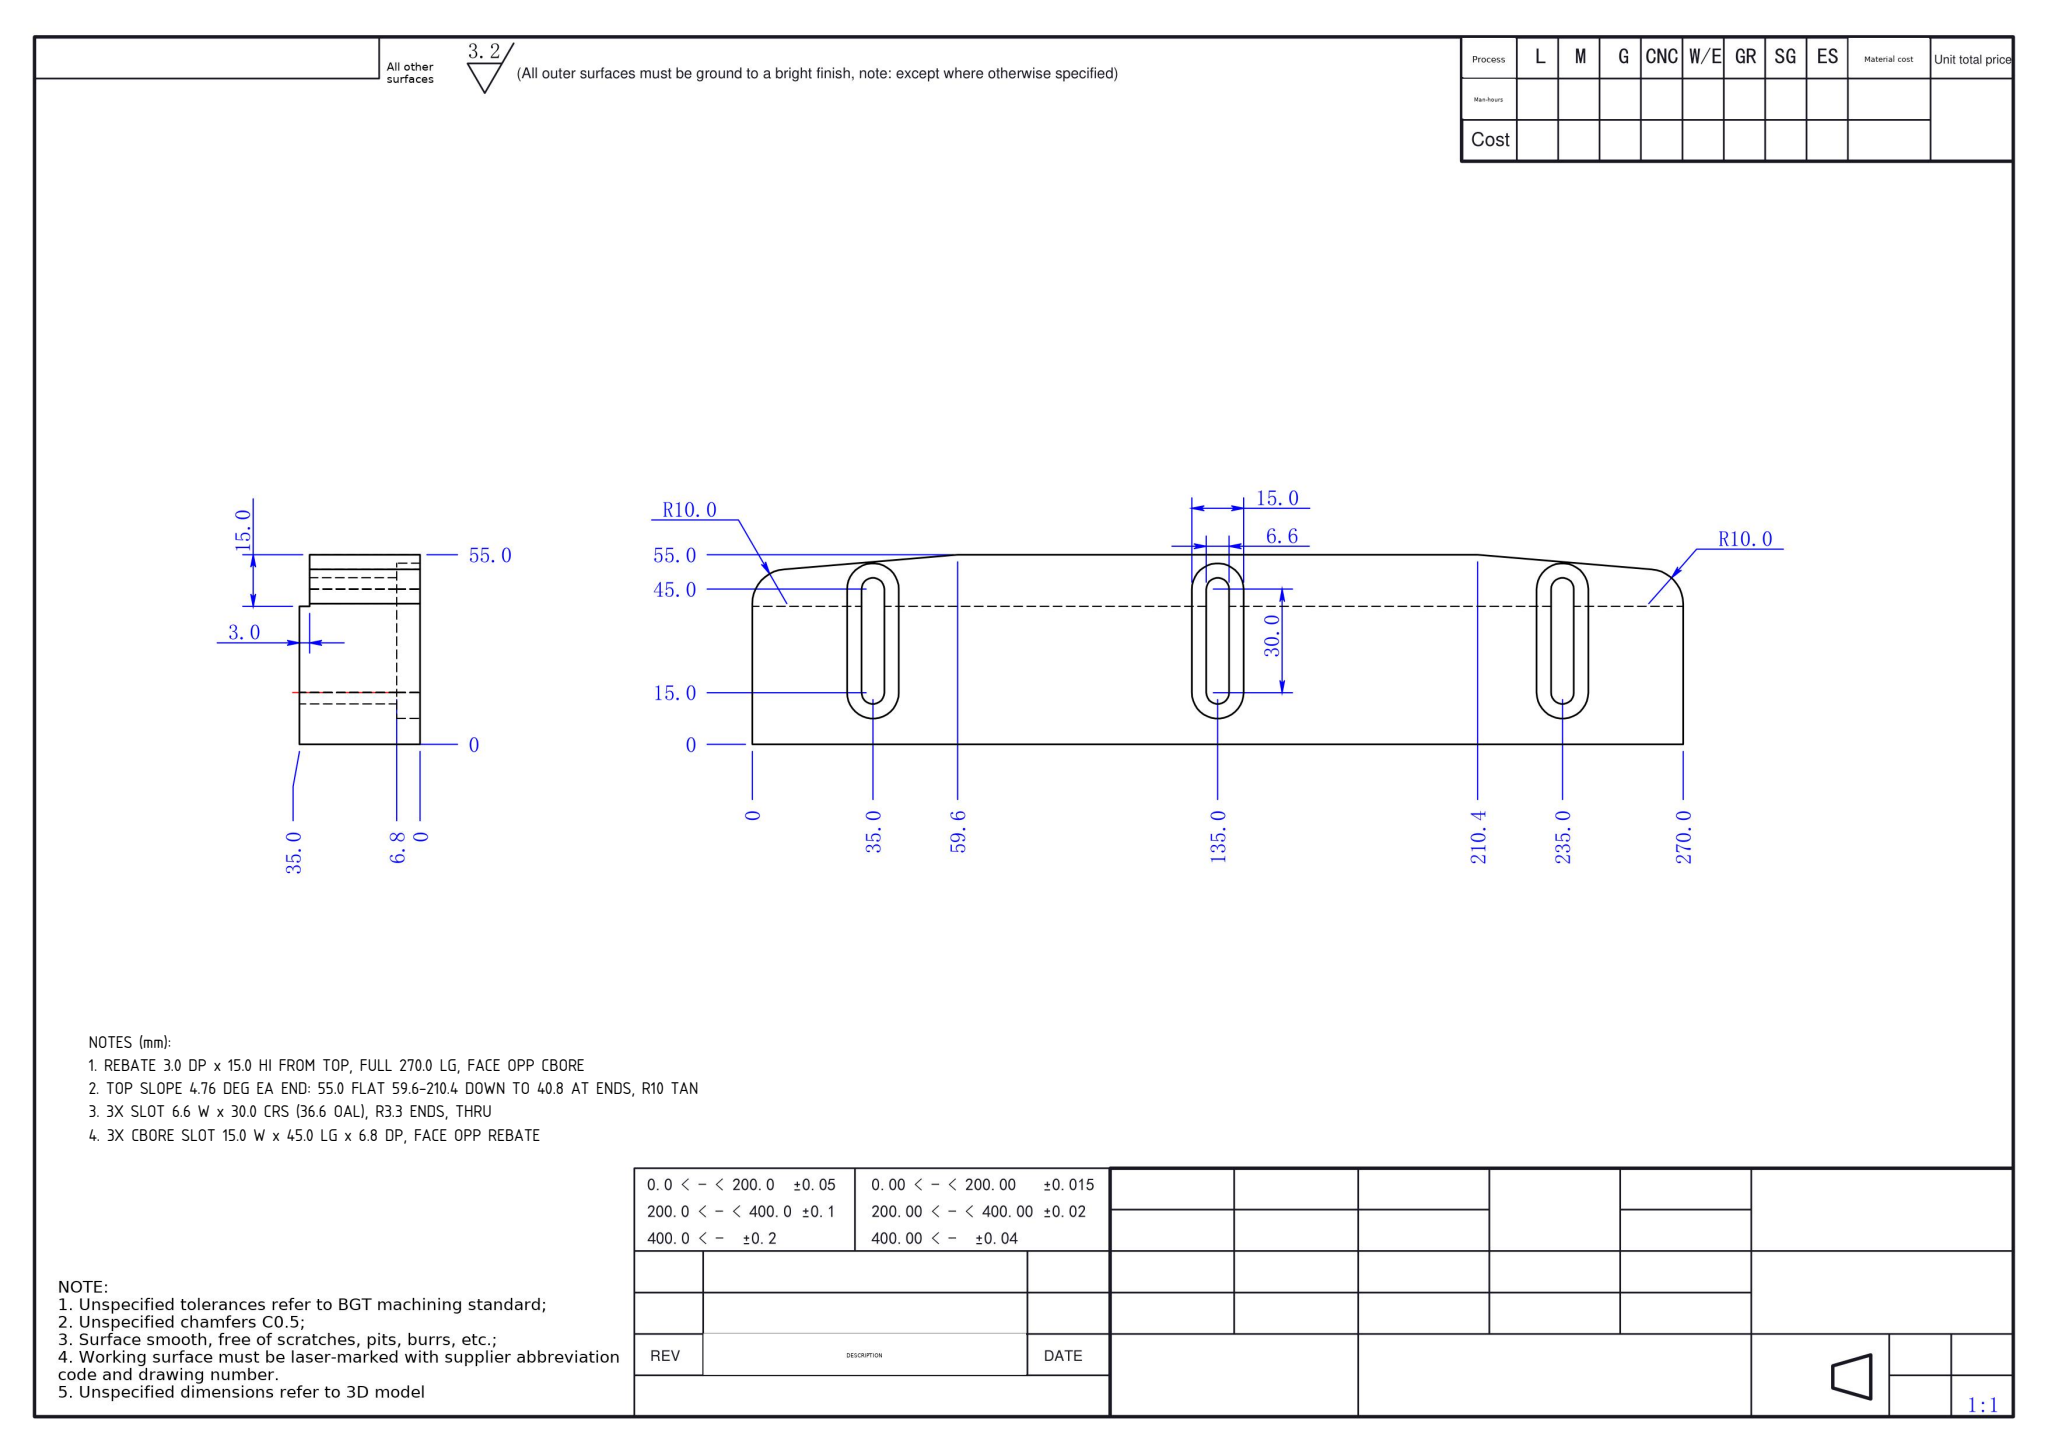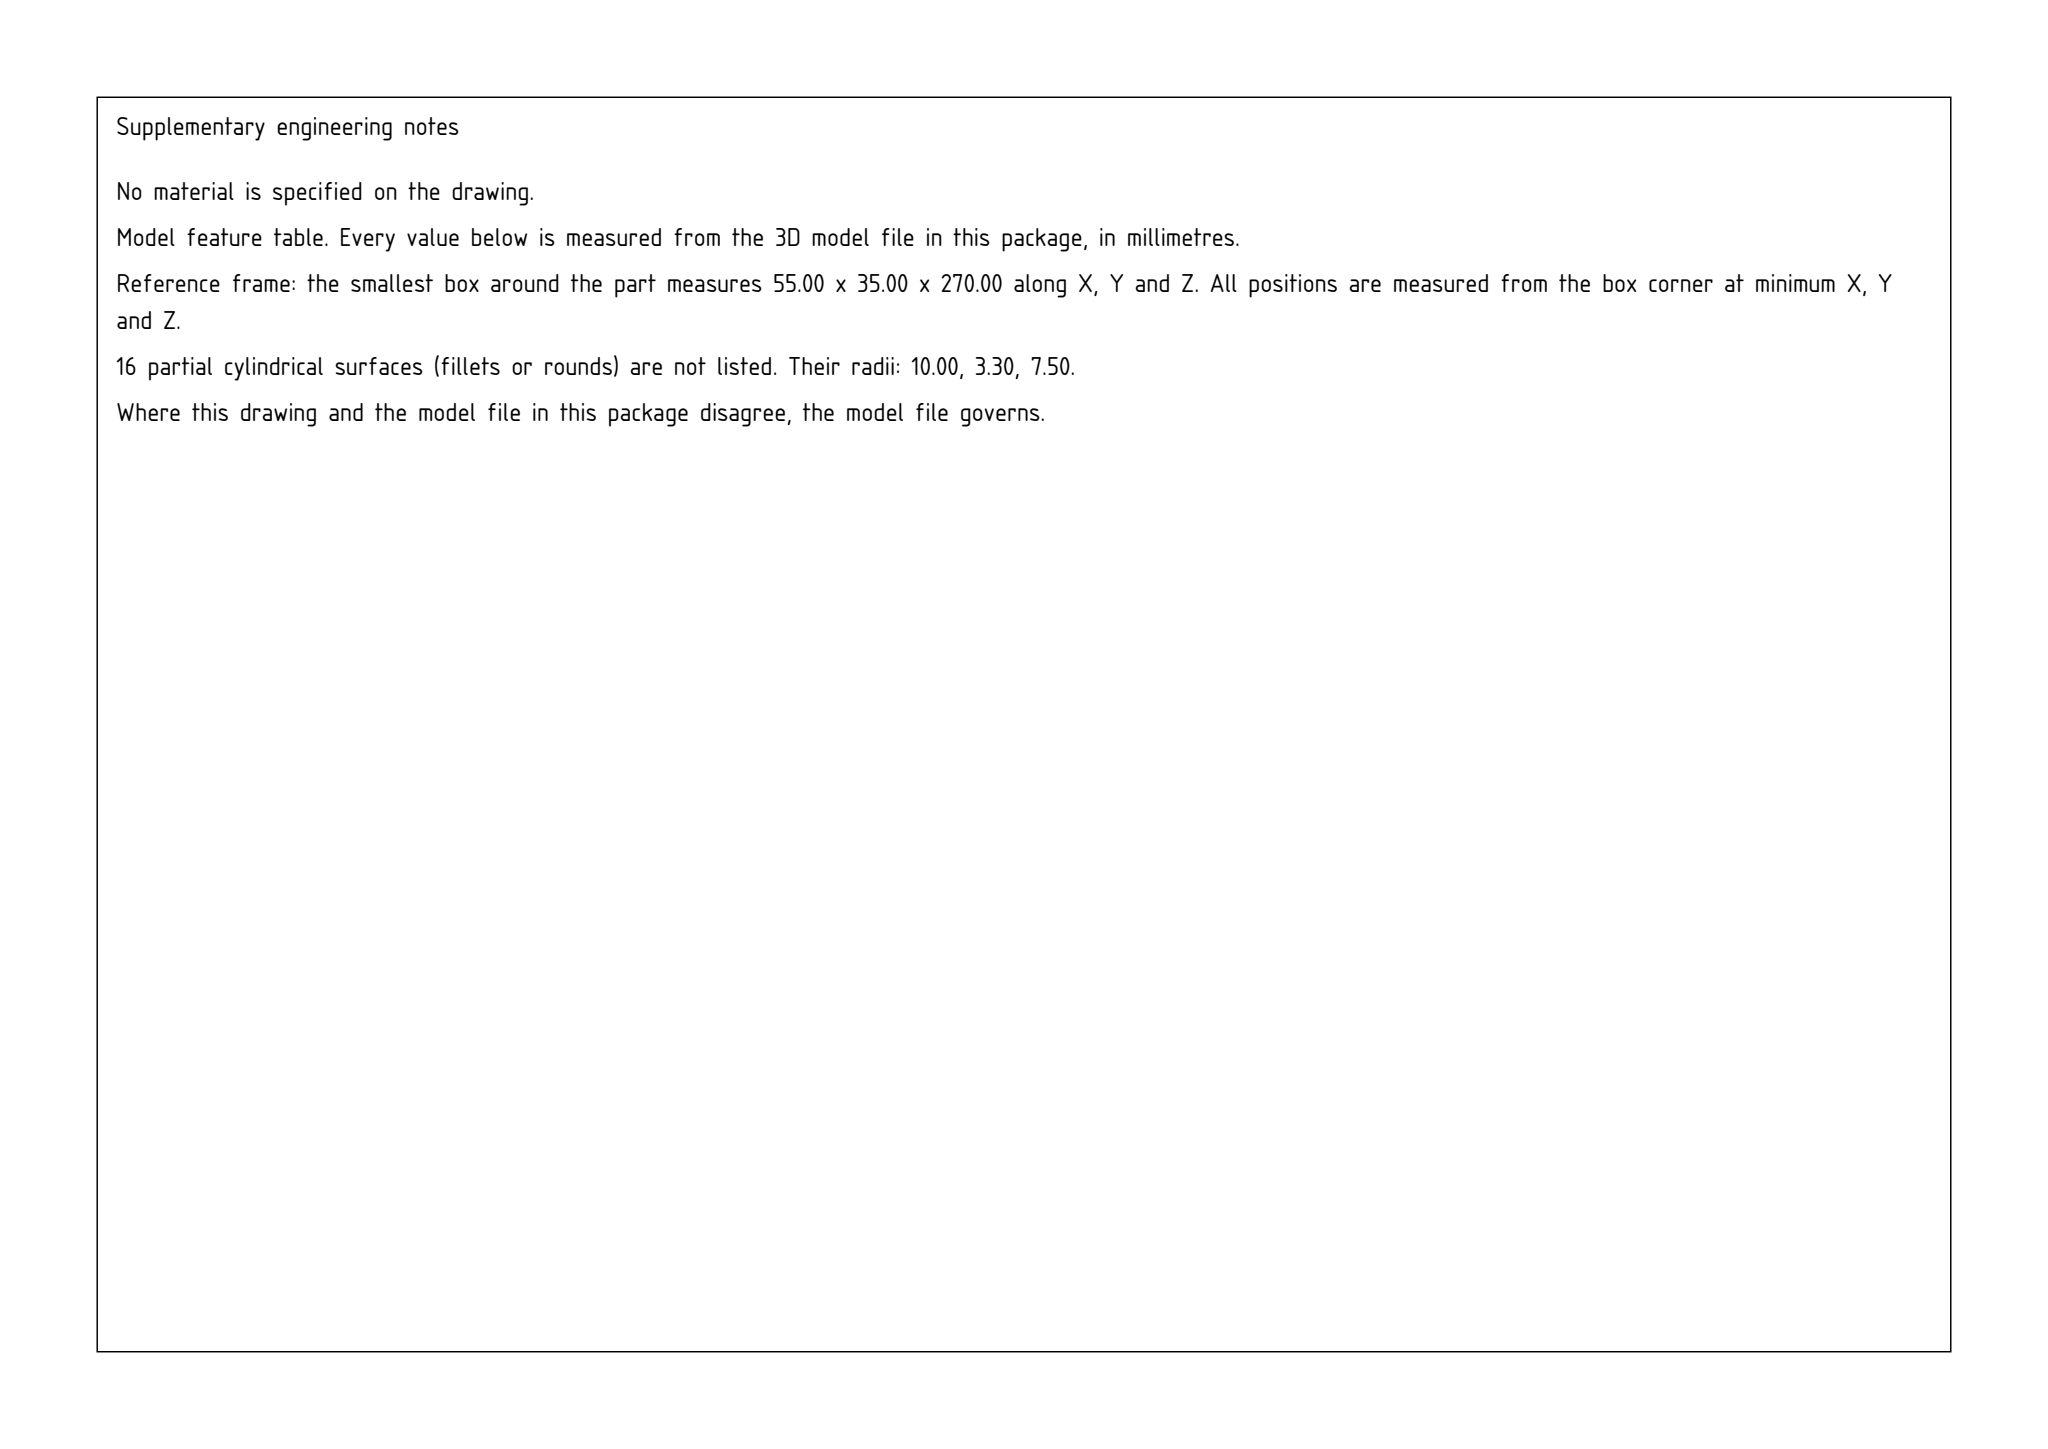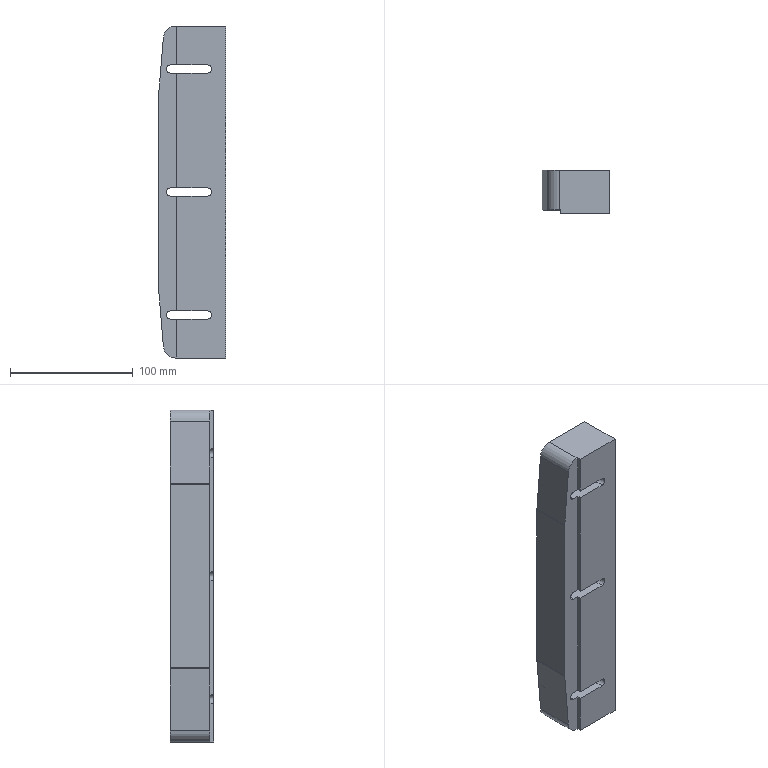Part | SolidWorks | mm | 1 solid | 50 faces | box 55 x 35 x 270 mm | volume 464892 mm3 | plane 28 | cylinder 22 | commonest cylinder face diameters 15 x9 6.6 x9 20 x4
Drawing notes:
REBATE 3.0 DP x 15.0 HI FROM TOP, FULL 270.0 LG, FACE OPP CBORE | from the solid: y planes 0/3.0 vs 28.2/35.0; x=15.0 planes (top 15 of 55 ht); runs full z=0-270; rebate region thk 32.0
TOP SLOPE 4.76 DEG EA END: 55.0 FLAT 59.6-210.4 DOWN TO 40.8 AT ENDS, R10 TAN | from the solid: R10 cyls (x10,z60.42)&(x10,z209.58) and (x14.2,z10)&(x14.2,z260); 55-14.2=40.8; atan(4.2/50.42)=4.76 deg
3X SLOT 6.6 W x 30.0 CRS (36.6 OAL), R3.3 ENDS, THRU | from the solid: O6.6 y-cyls at x=10 & x=40 (30 apart), z=35/135/235; z planes 31.7/38.3; lengths 25.2 & 28.2 = full remaining thk
3X CBORE SLOT 15.0 W x 45.0 LG x 6.8 DP, FACE OPP REBATE | from the solid: O15.0 y-cyls len 6.8 at x=10 & x=40, z=35/135/235; y planes 28.2 vs 35.0 face